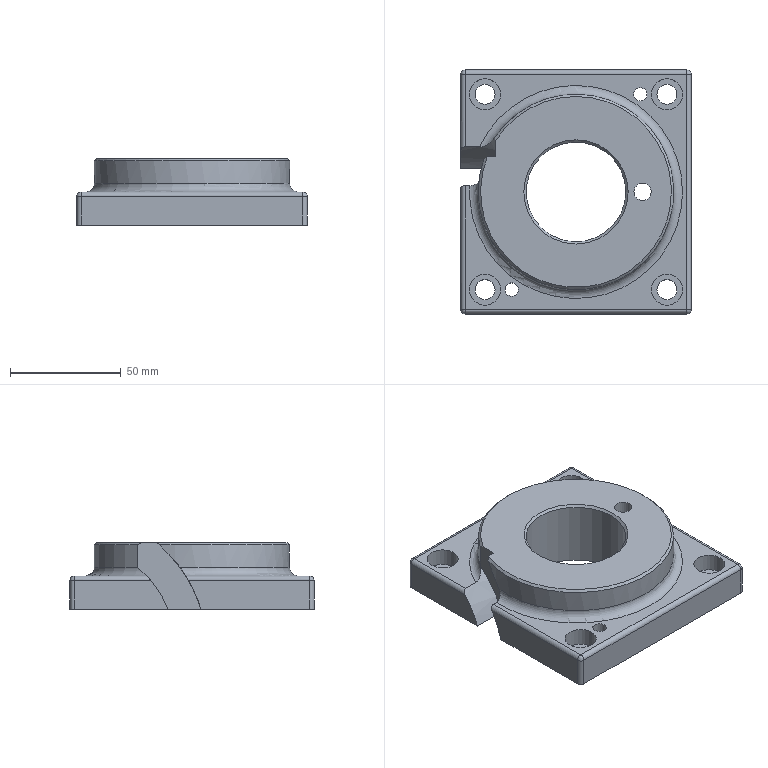Component | NX | DRILL_TEMPLATE | 1 solid | 44 faces | volume 201760 mm3 | cylinder 24 | plane 13 | sphere 4 | cone 2 | torus 1 | commonest cylinder face diameters 4 x9 9 x4 14 x4 6 x2 88 x1 7.8 x1 45 x1 100 x1